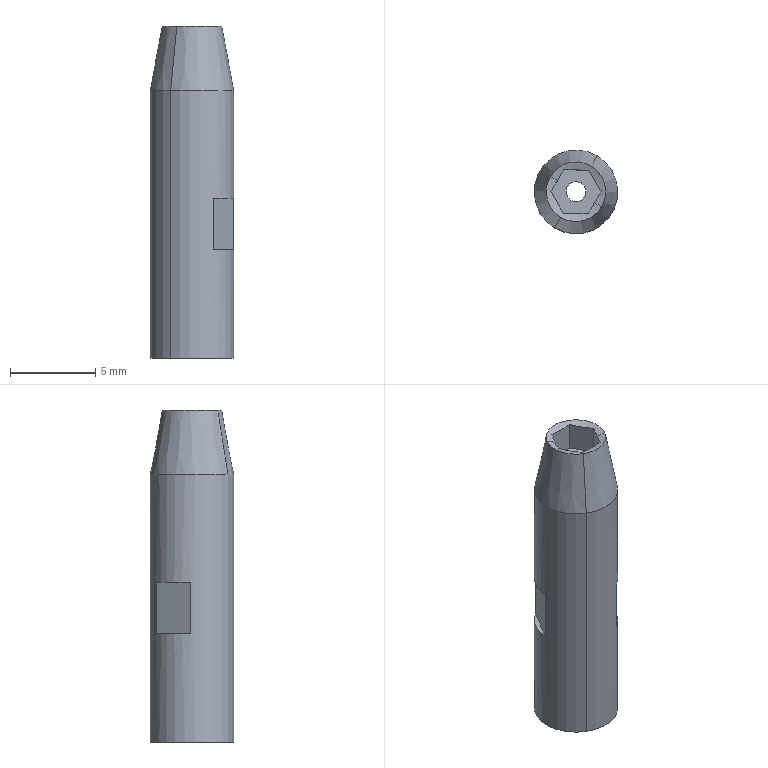Component | SolidWorks | PointedHead-2 | 1 solid | 24 faces | box 4.9 x 4.9 x 19.5 mm | volume 169 mm3 | plane 14 | cone 4 | cylinder 4 | sphere 2 | commonest cylinder face diameters 3.5 x2 4.9 x2
build123d program:
from build123d import *

# Parameters (mm, degrees)
SKETCH1_R                      = 2.45
EXTRUDE1_DEPTH                 = 19.5
CHAMFER1_SIZE                  = 0.7
CHAMFER1_SIZE2                 = 3.8
F_3_5_3_5_DIAMETER_HOLE1_D     = 3.5
F_3_5_3_5_DIAMETER_HOLE1_DEPTH = 17
F_3_5_3_5_DIAMETER_HOLE1_TIP   = 1.052
CUT_EXTRUDE1_DEPTH             = 1.8
CUT_EXTRUDE2_DEPTH             = 20.805
CUT_EXTRUDE2_DEPTH_BACK        = 20.805
SKETCH6_W                      = 3
SKETCH6_H                      = 0.3


with BuildPart() as part:
    # Sketch1 → Extrude1 (new body)
    with BuildSketch(Plane(origin=(0, 0, 0), x_dir=(0, 0, -1), z_dir=(1, 0, 0))):
        Circle(SKETCH1_R)
    extrude(amount=EXTRUDE1_DEPTH)

    # Chamfer1
    chamfer1_edges = [part.edges().sort_by_distance(p)[0] for p in [
        (0, 0, 2.45),
    ]]
    chamfer1_side = [part.faces().sort_by_distance(p)[0] for p in [
        (0, 0, 0),
    ]]
    chamfer(chamfer1_edges, length=CHAMFER1_SIZE, length2=CHAMFER1_SIZE2, reference=chamfer1_side[0])

    # 3.5 _3.5_ Diameter Hole1
    with Locations(Plane(origin=(19.5, 0, 0), x_dir=(0, 0, -1), z_dir=(1, 0, 0))):
        with Locations((0, 0)):
            Hole(F_3_5_3_5_DIAMETER_HOLE1_D / 2, depth=F_3_5_3_5_DIAMETER_HOLE1_DEPTH)
            with Locations((0, 0, -(F_3_5_3_5_DIAMETER_HOLE1_DEPTH + F_3_5_3_5_DIAMETER_HOLE1_TIP / 2))):  # 118° drill point
                Cone(0, F_3_5_3_5_DIAMETER_HOLE1_D / 2, F_3_5_3_5_DIAMETER_HOLE1_TIP, mode=Mode.SUBTRACT)

    # Sketch4 → Cut-Extrude1 (cut)
    with BuildSketch(Plane.ZY):
        Polygon((1.472, 0), (0.7361, 1.275), (-0.7361, 1.275), (-1.472, 0), (-0.7361, -1.275), (0.7361, -1.275), align=None)
    extrude(amount=-CUT_EXTRUDE1_DEPTH, mode=Mode.SUBTRACT)

    # Sketch5 → Cut-Revolve2 (revolve, cut)
    with BuildSketch(Plane.XY, mode=Mode.PRIVATE) as cut_revolve2_sk:
        with BuildLine():
            Line((0, 1.75), (0, 0))
            Line((0, 0), (0.3163, 0))
            ThreePointArc((0.3163, 0), (0.2366, 0.8892), (0, 1.75))
        make_face()
    revolve(cut_revolve2_sk.sketch.rotate(Axis((0, 0, 0), (-1, 0, 0)), 90), axis=Axis((0, 0, 0), (-1, 0, 0)), mode=Mode.SUBTRACT)

    # Sketch6 → Cut-Extrude2 (cut, two sides: drawn at the far end of the back side and taken through both)
    with BuildSketch(Plane.XY.offset(-CUT_EXTRUDE2_DEPTH_BACK)):
        with Locations((11.65, 2.3)):
            Rectangle(SKETCH6_W, SKETCH6_H)
        with Locations((11.65, -2.3)):
            Rectangle(SKETCH6_W, SKETCH6_H)
    extrude(amount=CUT_EXTRUDE2_DEPTH + CUT_EXTRUDE2_DEPTH_BACK, mode=Mode.SUBTRACT)


solid = part.part

# Placed as in the assembly
solid = solid.moved(Location((22.667, 79.622, -18.387), (90, -30.736, -90)))
STEP:
#1=CARTESIAN_POINT('',(0.8332,3.17,-0.7239));
#2=VERTEX_POINT('',#1);
#3=CARTESIAN_POINT('',(0.9276,3.194,-0.7239));
#4=VERTEX_POINT('',#3);
#5=CARTESIAN_POINT('',(0.8924,3.135,-0.7239));
#6=DIRECTION('',(-0.,0.,-1.));
#7=DIRECTION('',(-0.8595,0.5111,0.));
#8=AXIS2_PLACEMENT_3D('',#5,#6,#7);
#9=CIRCLE('',#8,0.0689);
#10=EDGE_CURVE('',#2,#4,#9,.T.);
#11=ORIENTED_EDGE('',*,*,#10,.F.);
#12=CARTESIAN_POINT('',(0.8493,3.16,-0.7298));
#13=VERTEX_POINT('',#12);
#14=CARTESIAN_POINT('',(0.8924,3.135,-0.5395));
#15=DIRECTION('',(-0.5111,-0.8595,0.));
#16=DIRECTION('',(0.8595,-0.5111,0.));
#17=AXIS2_PLACEMENT_3D('',#14,#15,#16);
#18=CIRCLE('',#17,0.1969);
#19=EDGE_CURVE('',#2,#13,#18,.T.);
#20=ORIENTED_EDGE('',*,*,#19,.T.);
#21=CARTESIAN_POINT('',(0.8641,3.185,-0.7276));
#22=VERTEX_POINT('',#21);
#23=CARTESIAN_POINT('',(0.8493,3.16,-0.5395));
#24=DIRECTION('',(-0.8595,0.5111,0.));
#25=DIRECTION('',(0.5111,0.8595,0.));
#26=AXIS2_PLACEMENT_3D('',#23,#24,#25);
#27=CIRCLE('',#26,0.1903);
#28=EDGE_CURVE('',#22,#13,#27,.T.);
#29=ORIENTED_EDGE('',*,*,#28,.F.);
#30=CARTESIAN_POINT('',(0.922,3.185,-0.7276));
#31=VERTEX_POINT('',#30);
#32=CARTESIAN_POINT('',(0.893,3.185,-0.5395));
#33=DIRECTION('',(0.01285,0.9999,-0.));
#34=DIRECTION('',(0.9999,-0.01285,-0.));
#35=AXIS2_PLACEMENT_3D('',#32,#33,#34);
#36=CIRCLE('',#35,0.1903);
#37=EDGE_CURVE('',#31,#22,#36,.T.);
#38=ORIENTED_EDGE('',*,*,#37,.F.);
#39=CARTESIAN_POINT('',(0.9504,3.134,-0.7276));
#40=VERTEX_POINT('',#39);
#41=CARTESIAN_POINT('',(0.9362,3.159,-0.5395));
#42=DIRECTION('',(0.8724,0.4888,-0.));
#43=DIRECTION('',(0.4888,-0.8724,0.));
#44=AXIS2_PLACEMENT_3D('',#41,#42,#43);
#45=CIRCLE('',#44,0.1903);
#46=EDGE_CURVE('',#40,#31,#45,.T.);
#47=ORIENTED_EDGE('',*,*,#46,.F.);
#48=CARTESIAN_POINT('',(0.9355,3.109,-0.7298));
#49=VERTEX_POINT('',#48);
#50=CARTESIAN_POINT('',(0.9355,3.109,-0.5395));
#51=DIRECTION('',(0.8595,-0.5111,-0.));
#52=DIRECTION('',(-0.5111,-0.8595,0.));
#53=AXIS2_PLACEMENT_3D('',#50,#51,#52);
#54=CIRCLE('',#53,0.1903);
#55=EDGE_CURVE('',#49,#40,#54,.T.);
#56=ORIENTED_EDGE('',*,*,#55,.F.);
#57=CARTESIAN_POINT('',(0.9516,3.1,-0.7239));
#58=VERTEX_POINT('',#57);
#59=CARTESIAN_POINT('',(0.8924,3.135,-0.5395));
#60=DIRECTION('',(0.5111,0.8595,-0.));
#61=DIRECTION('',(-0.8595,0.5111,0.));
#62=AXIS2_PLACEMENT_3D('',#59,#60,#61);
#63=CIRCLE('',#62,0.1969);
#64=EDGE_CURVE('',#58,#49,#63,.T.);
#65=ORIENTED_EDGE('',*,*,#64,.F.);
#66=CARTESIAN_POINT('',(0.8924,3.135,-0.7239));
#67=DIRECTION('',(-0.,0.,-1.));
#68=DIRECTION('',(-0.8595,0.5111,0.));
#69=AXIS2_PLACEMENT_3D('',#66,#67,#68);
#70=CIRCLE('',#69,0.0689);
#71=EDGE_CURVE('',#4,#58,#70,.T.);
#72=ORIENTED_EDGE('',*,*,#71,.F.);
#73=EDGE_LOOP('',(#11,#20,#29,#38,#47,#56,#65,#72));
#74=FACE_OUTER_BOUND('',#73,.T.);
#75=CARTESIAN_POINT('',(0.8924,3.135,-0.5395));
#76=DIRECTION('',(-0.5111,-0.8595,0.));
#77=DIRECTION('',(0.8595,-0.5111,-0.));
#78=AXIS2_PLACEMENT_3D('',#75,#76,#77);
#79=SPHERICAL_SURFACE('',#78,0.1969);
#80=ADVANCED_FACE('',(#74),#79,.F.);
#81=CARTESIAN_POINT('',(0.8806,3.115,-0.7948));
#82=VERTEX_POINT('',#81);
#83=CARTESIAN_POINT('',(0.9042,3.155,-0.7948));
#84=VERTEX_POINT('',#83);
#85=CARTESIAN_POINT('',(0.8924,3.135,-0.7948));
#86=DIRECTION('',(0.,-0.,1.));
#87=DIRECTION('',(-0.5111,-0.8595,0.));
#88=AXIS2_PLACEMENT_3D('',#85,#86,#87);
#89=CIRCLE('',#88,0.02303);
#90=EDGE_CURVE('',#82,#84,#89,.T.);
#91=ORIENTED_EDGE('',*,*,#90,.T.);
#92=CARTESIAN_POINT('',(0.9276,3.194,-0.8223));
#93=VERTEX_POINT('',#92);
#94=CARTESIAN_POINT('',(0.9276,3.194,-0.8223));
#95=DIRECTION('',(0.4381,0.7368,-0.515));
#96=VECTOR('',#95,39.37);
#97=LINE('',#94,#96);
#98=EDGE_CURVE('',#84,#93,#97,.T.);
#99=ORIENTED_EDGE('',*,*,#98,.T.);
#100=CARTESIAN_POINT('',(0.8572,3.076,-0.8223));
#101=VERTEX_POINT('',#100);
#102=CARTESIAN_POINT('',(0.8924,3.135,-0.8223));
#103=DIRECTION('',(-0.,0.,-1.));
#104=DIRECTION('',(-0.5111,-0.8595,0.));
#105=AXIS2_PLACEMENT_3D('',#102,#103,#104);
#106=CIRCLE('',#105,0.0689);
#107=EDGE_CURVE('',#93,#101,#106,.T.);
#108=ORIENTED_EDGE('',*,*,#107,.T.);
#109=CARTESIAN_POINT('',(0.8572,3.076,-0.8223));
#110=DIRECTION('',(-0.4381,-0.7368,-0.515));
#111=VECTOR('',#110,39.37);
#112=LINE('',#109,#111);
#113=EDGE_CURVE('',#82,#101,#112,.T.);
#114=ORIENTED_EDGE('',*,*,#113,.F.);
#115=EDGE_LOOP('',(#91,#99,#108,#114));
#116=FACE_OUTER_BOUND('',#115,.T.);
#117=CARTESIAN_POINT('',(0.8924,3.135,-0.8223));
#118=DIRECTION('',(-0.,0.,-1.));
#119=DIRECTION('',(-0.5111,-0.8595,0.));
#120=AXIS2_PLACEMENT_3D('',#117,#118,#119);
#121=CONICAL_SURFACE('',#120,0.0689,1.03);
#122=ADVANCED_FACE('',(#116),#121,.F.);
#123=ORIENTED_EDGE('',*,*,#107,.F.);
#124=CARTESIAN_POINT('',(0.9276,3.194,-1.492));
#125=VERTEX_POINT('',#124);
#126=CARTESIAN_POINT('',(0.9276,3.194,-1.492));
#127=DIRECTION('',(-0.,0.,-1.));
#128=VECTOR('',#127,39.37);
#129=LINE('',#126,#128);
#130=EDGE_CURVE('',#93,#125,#129,.T.);
#131=ORIENTED_EDGE('',*,*,#130,.T.);
#132=CARTESIAN_POINT('',(0.8572,3.076,-1.492));
#133=VERTEX_POINT('',#132);
#134=CARTESIAN_POINT('',(0.8924,3.135,-1.492));
#135=DIRECTION('',(-0.,0.,-1.));
#136=DIRECTION('',(-0.5111,-0.8595,0.));
#137=AXIS2_PLACEMENT_3D('',#134,#135,#136);
#138=CIRCLE('',#137,0.0689);
#139=EDGE_CURVE('',#125,#133,#138,.T.);
#140=ORIENTED_EDGE('',*,*,#139,.T.);
#141=CARTESIAN_POINT('',(0.8572,3.076,-1.492));
#142=DIRECTION('',(-0.,0.,-1.));
#143=VECTOR('',#142,39.37);
#144=LINE('',#141,#143);
#145=EDGE_CURVE('',#101,#133,#144,.T.);
#146=ORIENTED_EDGE('',*,*,#145,.F.);
#147=EDGE_LOOP('',(#123,#131,#140,#146));
#148=FACE_OUTER_BOUND('',#147,.T.);
#149=CARTESIAN_POINT('',(0.8924,3.135,-1.492));
#150=DIRECTION('',(-0.,0.,-1.));
#151=DIRECTION('',(-0.5111,-0.8595,0.));
#152=AXIS2_PLACEMENT_3D('',#149,#150,#151);
#153=CYLINDRICAL_SURFACE('',#152,0.0689);
#154=ADVANCED_FACE('',(#148),#153,.F.);
#155=CARTESIAN_POINT('',(0.8572,3.076,-0.7239));
#156=VERTEX_POINT('',#155);
#157=CARTESIAN_POINT('',(0.8924,3.135,-0.7239));
#158=DIRECTION('',(-0.,0.,-1.));
#159=DIRECTION('',(-0.8595,0.5111,0.));
#160=AXIS2_PLACEMENT_3D('',#157,#158,#159);
#161=CIRCLE('',#160,0.0689);
#162=EDGE_CURVE('',#156,#2,#161,.T.);
#163=ORIENTED_EDGE('',*,*,#162,.T.);
#164=ORIENTED_EDGE('',*,*,#10,.T.);
#165=CARTESIAN_POINT('',(0.9417,3.218,-0.8735));
#166=VERTEX_POINT('',#165);
#167=CARTESIAN_POINT('',(0.9417,3.218,-0.8735));
#168=DIRECTION('',(0.09259,0.1557,-0.9835));
#169=VECTOR('',#168,39.37);
#170=LINE('',#167,#169);
#171=EDGE_CURVE('',#4,#166,#170,.T.);
#172=ORIENTED_EDGE('',*,*,#171,.T.);
#173=CARTESIAN_POINT('',(0.8431,3.052,-0.8735));
#174=VERTEX_POINT('',#173);
#175=CARTESIAN_POINT('',(0.8924,3.135,-0.8735));
#176=DIRECTION('',(-0.,0.,-1.));
#177=DIRECTION('',(-0.5111,-0.8595,0.));
#178=AXIS2_PLACEMENT_3D('',#175,#176,#177);
#179=CIRCLE('',#178,0.09646);
#180=EDGE_CURVE('',#174,#166,#179,.T.);
#181=ORIENTED_EDGE('',*,*,#180,.F.);
#182=CARTESIAN_POINT('',(0.8431,3.052,-0.8735));
#183=DIRECTION('',(-0.09259,-0.1557,-0.9835));
#184=VECTOR('',#183,39.37);
#185=LINE('',#182,#184);
#186=EDGE_CURVE('',#156,#174,#185,.T.);
#187=ORIENTED_EDGE('',*,*,#186,.F.);
#188=EDGE_LOOP('',(#163,#164,#172,#181,#187));
#189=FACE_OUTER_BOUND('',#188,.T.);
#190=CARTESIAN_POINT('',(0.8924,3.135,-0.8735));
#191=DIRECTION('',(-0.,0.,-1.));
#192=DIRECTION('',(-0.5111,-0.8595,0.));
#193=AXIS2_PLACEMENT_3D('',#190,#191,#192);
#194=CONICAL_SURFACE('',#193,0.09646,0.1822);
#195=ADVANCED_FACE('',(#189),#194,.T.);
#196=CARTESIAN_POINT('',(0.796,3.138,-1.242));
#197=VERTEX_POINT('',#196);
#198=CARTESIAN_POINT('',(0.8433,3.218,-1.242));
#199=VERTEX_POINT('',#198);
#200=CARTESIAN_POINT('',(0.8924,3.135,-1.242));
#201=DIRECTION('',(-0.,0.,-1.));
#202=DIRECTION('',(-0.5111,-0.8595,0.));
#203=AXIS2_PLACEMENT_3D('',#200,#201,#202);
#204=CIRCLE('',#203,0.09646);
#205=EDGE_CURVE('',#197,#199,#204,.T.);
#206=ORIENTED_EDGE('',*,*,#205,.T.);
#207=CARTESIAN_POINT('',(0.8433,3.218,-1.123));
#208=VERTEX_POINT('',#207);
#209=CARTESIAN_POINT('',(0.8433,3.218,-1.492));
#210=DIRECTION('',(0.,-0.,1.));
#211=VECTOR('',#210,39.37);
#212=LINE('',#209,#211);
#213=EDGE_CURVE('',#199,#208,#212,.T.);
#214=ORIENTED_EDGE('',*,*,#213,.T.);
#215=CARTESIAN_POINT('',(0.796,3.138,-1.123));
#216=VERTEX_POINT('',#215);
#217=CARTESIAN_POINT('',(0.8924,3.135,-1.123));
#218=DIRECTION('',(0.,-0.,1.));
#219=DIRECTION('',(0.5111,0.8595,0.));
#220=AXIS2_PLACEMENT_3D('',#217,#218,#219);
#221=CIRCLE('',#220,0.09646);
#222=EDGE_CURVE('',#208,#216,#221,.T.);
#223=ORIENTED_EDGE('',*,*,#222,.T.);
#224=CARTESIAN_POINT('',(0.796,3.138,-1.492));
#225=DIRECTION('',(-0.,0.,-1.));
#226=VECTOR('',#225,39.37);
#227=LINE('',#224,#226);
#228=EDGE_CURVE('',#216,#197,#227,.T.);
#229=ORIENTED_EDGE('',*,*,#228,.T.);
#230=EDGE_LOOP('',(#206,#214,#223,#229));
#231=FACE_BOUND('',#230,.T.);
#232=CARTESIAN_POINT('',(0.8431,3.052,-1.492));
#233=VERTEX_POINT('',#232);
#234=CARTESIAN_POINT('',(0.9417,3.218,-1.492));
#235=VERTEX_POINT('',#234);
#236=CARTESIAN_POINT('',(0.8924,3.135,-1.492));
#237=DIRECTION('',(-0.,0.,-1.));
#238=DIRECTION('',(-0.5111,-0.8595,0.));
#239=AXIS2_PLACEMENT_3D('',#236,#237,#238);
#240=CIRCLE('',#239,0.09646);
#241=EDGE_CURVE('',#233,#235,#240,.T.);
#242=ORIENTED_EDGE('',*,*,#241,.F.);
#243=CARTESIAN_POINT('',(0.8431,3.052,-1.492));
#244=DIRECTION('',(0.,-0.,1.));
#245=VECTOR('',#244,39.37);
#246=LINE('',#243,#245);
#247=EDGE_CURVE('',#233,#174,#246,.T.);
#248=ORIENTED_EDGE('',*,*,#247,.T.);
#249=ORIENTED_EDGE('',*,*,#180,.T.);
#250=CARTESIAN_POINT('',(0.9417,3.218,-1.492));
#251=DIRECTION('',(0.,-0.,1.));
#252=VECTOR('',#251,39.37);
#253=LINE('',#250,#252);
#254=EDGE_CURVE('',#235,#166,#253,.T.);
#255=ORIENTED_EDGE('',*,*,#254,.F.);
#256=EDGE_LOOP('',(#242,#248,#249,#255));
#257=FACE_OUTER_BOUND('',#256,.T.);
#258=CARTESIAN_POINT('',(0.8924,3.135,-1.492));
#259=DIRECTION('',(0.,-0.,1.));
#260=DIRECTION('',(0.5111,0.8595,0.));
#261=AXIS2_PLACEMENT_3D('',#258,#259,#260);
#262=CYLINDRICAL_SURFACE('',#261,0.09646);
#263=ADVANCED_FACE('',(#231,#257),#262,.T.);
#264=ORIENTED_EDGE('',*,*,#247,.F.);
#265=CARTESIAN_POINT('',(0.8924,3.135,-1.492));
#266=DIRECTION('',(-0.,0.,-1.));
#267=DIRECTION('',(-0.5111,-0.8595,0.));
#268=AXIS2_PLACEMENT_3D('',#265,#266,#267);
#269=CIRCLE('',#268,0.09646);
#270=EDGE_CURVE('',#235,#233,#269,.T.);
#271=ORIENTED_EDGE('',*,*,#270,.F.);
#272=ORIENTED_EDGE('',*,*,#254,.T.);
#273=CARTESIAN_POINT('',(0.8924,3.135,-0.8735));
#274=DIRECTION('',(-0.,0.,-1.));
#275=DIRECTION('',(-0.5111,-0.8595,0.));
#276=AXIS2_PLACEMENT_3D('',#273,#274,#275);
#277=CIRCLE('',#276,0.09646);
#278=EDGE_CURVE('',#166,#174,#277,.T.);
#279=ORIENTED_EDGE('',*,*,#278,.T.);
#280=EDGE_LOOP('',(#264,#271,#272,#279));
#281=FACE_OUTER_BOUND('',#280,.T.);
#282=CARTESIAN_POINT('',(0.9888,3.131,-1.123));
#283=VERTEX_POINT('',#282);
#284=CARTESIAN_POINT('',(0.9888,3.131,-1.242));
#285=VERTEX_POINT('',#284);
#286=CARTESIAN_POINT('',(0.9888,3.131,-1.492));
#287=DIRECTION('',(-0.,0.,-1.));
#288=VECTOR('',#287,39.37);
#289=LINE('',#286,#288);
#290=EDGE_CURVE('',#283,#285,#289,.T.);
#291=ORIENTED_EDGE('',*,*,#290,.T.);
#292=CARTESIAN_POINT('',(0.9415,3.052,-1.242));
#293=VERTEX_POINT('',#292);
#294=CARTESIAN_POINT('',(0.8924,3.135,-1.242));
#295=DIRECTION('',(-0.,0.,-1.));
#296=DIRECTION('',(-0.8595,0.5111,0.));
#297=AXIS2_PLACEMENT_3D('',#294,#295,#296);
#298=CIRCLE('',#297,0.09646);
#299=EDGE_CURVE('',#285,#293,#298,.T.);
#300=ORIENTED_EDGE('',*,*,#299,.T.);
#301=CARTESIAN_POINT('',(0.9415,3.052,-1.123));
#302=VERTEX_POINT('',#301);
#303=CARTESIAN_POINT('',(0.9415,3.052,-1.492));
#304=DIRECTION('',(0.,-0.,1.));
#305=VECTOR('',#304,39.37);
#306=LINE('',#303,#305);
#307=EDGE_CURVE('',#293,#302,#306,.T.);
#308=ORIENTED_EDGE('',*,*,#307,.T.);
#309=CARTESIAN_POINT('',(0.8924,3.135,-1.123));
#310=DIRECTION('',(-0.,0.,1.));
#311=DIRECTION('',(0.8595,-0.5111,0.));
#312=AXIS2_PLACEMENT_3D('',#309,#310,#311);
#313=CIRCLE('',#312,0.09646);
#314=EDGE_CURVE('',#302,#283,#313,.T.);
#315=ORIENTED_EDGE('',*,*,#314,.T.);
#316=EDGE_LOOP('',(#291,#300,#308,#315));
#317=FACE_BOUND('',#316,.T.);
#318=CARTESIAN_POINT('',(0.8924,3.135,-1.492));
#319=DIRECTION('',(0.,-0.,1.));
#320=DIRECTION('',(0.5111,0.8595,0.));
#321=AXIS2_PLACEMENT_3D('',#318,#319,#320);
#322=CYLINDRICAL_SURFACE('',#321,0.09646);
#323=ADVANCED_FACE('',(#281,#317),#322,.T.);
#324=CARTESIAN_POINT('',(0.8924,3.135,-1.492));
#325=DIRECTION('',(-0.,0.,-1.));
#326=DIRECTION('',(-0.5111,-0.8595,0.));
#327=AXIS2_PLACEMENT_3D('',#324,#325,#326);
#328=CIRCLE('',#327,0.0689);
#329=EDGE_CURVE('',#133,#125,#328,.T.);
#330=ORIENTED_EDGE('',*,*,#329,.F.);
#331=ORIENTED_EDGE('',*,*,#139,.F.);
#332=EDGE_LOOP('',(#330,#331));
#333=FACE_BOUND('',#332,.T.);
#334=ORIENTED_EDGE('',*,*,#270,.T.);
#335=ORIENTED_EDGE('',*,*,#241,.T.);
#336=EDGE_LOOP('',(#334,#335));
#337=FACE_OUTER_BOUND('',#336,.T.);
#338=CARTESIAN_POINT('',(0.8924,3.135,-1.492));
#339=DIRECTION('',(-0.,0.,-1.));
#340=DIRECTION('',(-0.5111,-0.8595,0.));
#341=AXIS2_PLACEMENT_3D('',#338,#339,#340);
#342=PLANE('',#341);
#343=ADVANCED_FACE('',(#333,#337),#342,.T.);
#344=ORIENTED_EDGE('',*,*,#171,.F.);
#345=ORIENTED_EDGE('',*,*,#71,.T.);
#346=CARTESIAN_POINT('',(0.8924,3.135,-0.7239));
#347=DIRECTION('',(-0.,0.,-1.));
#348=DIRECTION('',(-0.8595,0.5111,0.));
#349=AXIS2_PLACEMENT_3D('',#346,#347,#348);
#350=CIRCLE('',#349,0.0689);
#351=EDGE_CURVE('',#58,#156,#350,.T.);
#352=ORIENTED_EDGE('',*,*,#351,.T.);
#353=ORIENTED_EDGE('',*,*,#186,.T.);
#354=ORIENTED_EDGE('',*,*,#278,.F.);
#355=EDGE_LOOP('',(#344,#345,#352,#353,#354));
#356=FACE_OUTER_BOUND('',#355,.T.);
#357=CARTESIAN_POINT('',(0.8924,3.135,-0.8735));
#358=DIRECTION('',(-0.,0.,-1.));
#359=DIRECTION('',(-0.5111,-0.8595,0.));
#360=AXIS2_PLACEMENT_3D('',#357,#358,#359);
#361=CONICAL_SURFACE('',#360,0.09646,0.1822);
#362=ADVANCED_FACE('',(#356),#361,.T.);
#363=ORIENTED_EDGE('',*,*,#130,.F.);
#364=CARTESIAN_POINT('',(0.8924,3.135,-0.8223));
#365=DIRECTION('',(-0.,0.,-1.));
#366=DIRECTION('',(-0.5111,-0.8595,0.));
#367=AXIS2_PLACEMENT_3D('',#364,#365,#366);
#368=CIRCLE('',#367,0.0689);
#369=EDGE_CURVE('',#101,#93,#368,.T.);
#370=ORIENTED_EDGE('',*,*,#369,.F.);
#371=ORIENTED_EDGE('',*,*,#145,.T.);
#372=ORIENTED_EDGE('',*,*,#329,.T.);
#373=EDGE_LOOP('',(#363,#370,#371,#372));
#374=FACE_OUTER_BOUND('',#373,.T.);
#375=CARTESIAN_POINT('',(0.8924,3.135,-1.492));
#376=DIRECTION('',(-0.,0.,-1.));
#377=DIRECTION('',(-0.5111,-0.8595,0.));
#378=AXIS2_PLACEMENT_3D('',#375,#376,#377);
#379=CYLINDRICAL_SURFACE('',#378,0.0689);
#380=ADVANCED_FACE('',(#374),#379,.F.);
#381=ORIENTED_EDGE('',*,*,#98,.F.);
#382=CARTESIAN_POINT('',(0.8924,3.135,-0.7948));
#383=DIRECTION('',(0.,-0.,1.));
#384=DIRECTION('',(-0.5111,-0.8595,0.));
#385=AXIS2_PLACEMENT_3D('',#382,#383,#384);
#386=CIRCLE('',#385,0.02303);
#387=EDGE_CURVE('',#84,#82,#386,.T.);
#388=ORIENTED_EDGE('',*,*,#387,.T.);
#389=ORIENTED_EDGE('',*,*,#113,.T.);
#390=ORIENTED_EDGE('',*,*,#369,.T.);
#391=EDGE_LOOP('',(#381,#388,#389,#390));
#392=FACE_OUTER_BOUND('',#391,.T.);
#393=CARTESIAN_POINT('',(0.8924,3.135,-0.8223));
#394=DIRECTION('',(-0.,0.,-1.));
#395=DIRECTION('',(-0.5111,-0.8595,0.));
#396=AXIS2_PLACEMENT_3D('',#393,#394,#395);
#397=CONICAL_SURFACE('',#396,0.0689,1.03);
#398=ADVANCED_FACE('',(#392),#397,.F.);
#399=CARTESIAN_POINT('',(0.9504,3.134,-0.7948));
#400=VERTEX_POINT('',#399);
#401=CARTESIAN_POINT('',(0.922,3.185,-0.7948));
#402=VERTEX_POINT('',#401);
#403=CARTESIAN_POINT('',(0.9504,3.134,-0.7948));
#404=DIRECTION('',(-0.4888,0.8724,0.));
#405=VECTOR('',#404,39.37);
#406=LINE('',#403,#405);
#407=EDGE_CURVE('',#400,#402,#406,.T.);
#408=ORIENTED_EDGE('',*,*,#407,.T.);
#409=CARTESIAN_POINT('',(0.8641,3.185,-0.7948));
#410=VERTEX_POINT('',#409);
#411=CARTESIAN_POINT('',(0.922,3.185,-0.7948));
#412=DIRECTION('',(-0.9999,0.01285,0.));
#413=VECTOR('',#412,39.37);
#414=LINE('',#411,#413);
#415=EDGE_CURVE('',#402,#410,#414,.T.);
#416=ORIENTED_EDGE('',*,*,#415,.T.);
#417=CARTESIAN_POINT('',(0.8344,3.135,-0.7948));
#418=VERTEX_POINT('',#417);
#419=CARTESIAN_POINT('',(0.8641,3.185,-0.7948));
#420=DIRECTION('',(-0.5111,-0.8595,0.));
#421=VECTOR('',#420,39.37);
#422=LINE('',#419,#421);
#423=EDGE_CURVE('',#410,#418,#422,.T.);
#424=ORIENTED_EDGE('',*,*,#423,.T.);
#425=CARTESIAN_POINT('',(0.8628,3.085,-0.7948));
#426=VERTEX_POINT('',#425);
#427=CARTESIAN_POINT('',(0.8344,3.135,-0.7948));
#428=DIRECTION('',(0.4888,-0.8724,-0.));
#429=VECTOR('',#428,39.37);
#430=LINE('',#427,#429);
#431=EDGE_CURVE('',#418,#426,#430,.T.);
#432=ORIENTED_EDGE('',*,*,#431,.T.);
#433=CARTESIAN_POINT('',(0.9207,3.084,-0.7948));
#434=VERTEX_POINT('',#433);
#435=CARTESIAN_POINT('',(0.8628,3.085,-0.7948));
#436=DIRECTION('',(0.9999,-0.01285,-0.));
#437=VECTOR('',#436,39.37);
#438=LINE('',#435,#437);
#439=EDGE_CURVE('',#426,#434,#438,.T.);
#440=ORIENTED_EDGE('',*,*,#439,.T.);
#441=CARTESIAN_POINT('',(0.9207,3.084,-0.7948));
#442=DIRECTION('',(0.5111,0.8595,-0.));
#443=VECTOR('',#442,39.37);
#444=LINE('',#441,#443);
#445=EDGE_CURVE('',#434,#400,#444,.T.);
#446=ORIENTED_EDGE('',*,*,#445,.T.);
#447=EDGE_LOOP('',(#408,#416,#424,#432,#440,#446));
#448=FACE_OUTER_BOUND('',#447,.T.);
#449=ORIENTED_EDGE('',*,*,#90,.F.);
#450=ORIENTED_EDGE('',*,*,#387,.F.);
#451=EDGE_LOOP('',(#449,#450));
#452=FACE_BOUND('',#451,.T.);
#453=CARTESIAN_POINT('',(0.9504,3.134,-0.7948));
#454=DIRECTION('',(-0.,0.,-1.));
#455=DIRECTION('',(-0.5111,-0.8595,0.));
#456=AXIS2_PLACEMENT_3D('',#453,#454,#455);
#457=PLANE('',#456);
#458=ADVANCED_FACE('',(#448,#452),#457,.F.);
#459=CARTESIAN_POINT('',(0.9504,3.134,-0.7948));
#460=DIRECTION('',(0.,-0.,1.));
#461=VECTOR('',#460,39.37);
#462=LINE('',#459,#461);
#463=EDGE_CURVE('',#400,#40,#462,.T.);
#464=ORIENTED_EDGE('',*,*,#463,.T.);
#465=ORIENTED_EDGE('',*,*,#46,.T.);
#466=CARTESIAN_POINT('',(0.922,3.185,-0.7948));
#467=DIRECTION('',(0.,-0.,1.));
#468=VECTOR('',#467,39.37);
#469=LINE('',#466,#468);
#470=EDGE_CURVE('',#402,#31,#469,.T.);
#471=ORIENTED_EDGE('',*,*,#470,.F.);
#472=ORIENTED_EDGE('',*,*,#407,.F.);
#473=EDGE_LOOP('',(#464,#465,#471,#472));
#474=FACE_OUTER_BOUND('',#473,.T.);
#475=CARTESIAN_POINT('',(0.9504,3.134,-0.7948));
#476=DIRECTION('',(0.8724,0.4888,-0.));
#477=DIRECTION('',(0.4888,-0.8724,-0.));
#478=AXIS2_PLACEMENT_3D('',#475,#476,#477);
#479=PLANE('',#478);
#480=ADVANCED_FACE('',(#474),#479,.F.);
#481=CARTESIAN_POINT('',(0.9207,3.084,-0.7276));
#482=VERTEX_POINT('',#481);
#483=CARTESIAN_POINT('',(0.9207,3.084,-0.7948));
#484=DIRECTION('',(0.,-0.,1.));
#485=VECTOR('',#484,39.37);
#486=LINE('',#483,#485);
#487=EDGE_CURVE('',#434,#482,#486,.T.);
#488=ORIENTED_EDGE('',*,*,#487,.T.);
#489=CARTESIAN_POINT('',(0.9355,3.109,-0.5395));
#490=DIRECTION('',(0.8595,-0.5111,-0.));
#491=DIRECTION('',(-0.5111,-0.8595,0.));
#492=AXIS2_PLACEMENT_3D('',#489,#490,#491);
#493=CIRCLE('',#492,0.1903);
#494=EDGE_CURVE('',#482,#49,#493,.T.);
#495=ORIENTED_EDGE('',*,*,#494,.T.);
#496=ORIENTED_EDGE('',*,*,#55,.T.);
#497=ORIENTED_EDGE('',*,*,#463,.F.);
#498=ORIENTED_EDGE('',*,*,#445,.F.);
#499=EDGE_LOOP('',(#488,#495,#496,#497,#498));
#500=FACE_OUTER_BOUND('',#499,.T.);
#501=CARTESIAN_POINT('',(0.9207,3.084,-0.7948));
#502=DIRECTION('',(0.8595,-0.5111,-0.));
#503=DIRECTION('',(-0.5111,-0.8595,0.));
#504=AXIS2_PLACEMENT_3D('',#501,#502,#503);
#505=PLANE('',#504);
#506=ADVANCED_FACE('',(#500),#505,.F.);
#507=CARTESIAN_POINT('',(0.8628,3.085,-0.7276));
#508=VERTEX_POINT('',#507);
#509=CARTESIAN_POINT('',(0.8628,3.085,-0.7948));
#510=DIRECTION('',(0.,-0.,1.));
#511=VECTOR('',#510,39.37);
#512=LINE('',#509,#511);
#513=EDGE_CURVE('',#426,#508,#512,.T.);
#514=ORIENTED_EDGE('',*,*,#513,.T.);
#515=CARTESIAN_POINT('',(0.8918,3.085,-0.5395));
#516=DIRECTION('',(-0.01285,-0.9999,0.));
#517=DIRECTION('',(-0.9999,0.01285,0.));
#518=AXIS2_PLACEMENT_3D('',#515,#516,#517);
#519=CIRCLE('',#518,0.1903);
#520=EDGE_CURVE('',#508,#482,#519,.T.);
#521=ORIENTED_EDGE('',*,*,#520,.T.);
#522=ORIENTED_EDGE('',*,*,#487,.F.);
#523=ORIENTED_EDGE('',*,*,#439,.F.);
#524=EDGE_LOOP('',(#514,#521,#522,#523));
#525=FACE_OUTER_BOUND('',#524,.T.);
#526=CARTESIAN_POINT('',(0.8628,3.085,-0.7948));
#527=DIRECTION('',(-0.01285,-0.9999,0.));
#528=DIRECTION('',(-0.9999,0.01285,0.));
#529=AXIS2_PLACEMENT_3D('',#526,#527,#528);
#530=PLANE('',#529);
#531=ADVANCED_FACE('',(#525),#530,.F.);
#532=CARTESIAN_POINT('',(0.8344,3.135,-0.7276));
#533=VERTEX_POINT('',#532);
#534=CARTESIAN_POINT('',(0.8344,3.135,-0.7948));
#535=DIRECTION('',(0.,-0.,1.));
#536=VECTOR('',#535,39.37);
#537=LINE('',#534,#536);
#538=EDGE_CURVE('',#418,#533,#537,.T.);
#539=ORIENTED_EDGE('',*,*,#538,.T.);
#540=CARTESIAN_POINT('',(0.8486,3.11,-0.5395));
#541=DIRECTION('',(-0.8724,-0.4888,0.));
#542=DIRECTION('',(-0.4888,0.8724,0.));
#543=AXIS2_PLACEMENT_3D('',#540,#541,#542);
#544=CIRCLE('',#543,0.1903);
#545=EDGE_CURVE('',#533,#508,#544,.T.);
#546=ORIENTED_EDGE('',*,*,#545,.T.);
#547=ORIENTED_EDGE('',*,*,#513,.F.);
#548=ORIENTED_EDGE('',*,*,#431,.F.);
#549=EDGE_LOOP('',(#539,#546,#547,#548));
#550=FACE_OUTER_BOUND('',#549,.T.);
#551=CARTESIAN_POINT('',(0.8344,3.135,-0.7948));
#552=DIRECTION('',(-0.8724,-0.4888,0.));
#553=DIRECTION('',(-0.4888,0.8724,0.));
#554=AXIS2_PLACEMENT_3D('',#551,#552,#553);
#555=PLANE('',#554);
#556=ADVANCED_FACE('',(#550),#555,.F.);
#557=CARTESIAN_POINT('',(0.8641,3.185,-0.7948));
#558=DIRECTION('',(0.,-0.,1.));
#559=VECTOR('',#558,39.37);
#560=LINE('',#557,#559);
#561=EDGE_CURVE('',#410,#22,#560,.T.);
#562=ORIENTED_EDGE('',*,*,#561,.T.);
#563=ORIENTED_EDGE('',*,*,#28,.T.);
#564=CARTESIAN_POINT('',(0.8493,3.16,-0.5395));
#565=DIRECTION('',(-0.8595,0.5111,0.));
#566=DIRECTION('',(0.5111,0.8595,0.));
#567=AXIS2_PLACEMENT_3D('',#564,#565,#566);
#568=CIRCLE('',#567,0.1903);
#569=EDGE_CURVE('',#13,#533,#568,.T.);
#570=ORIENTED_EDGE('',*,*,#569,.T.);
#571=ORIENTED_EDGE('',*,*,#538,.F.);
#572=ORIENTED_EDGE('',*,*,#423,.F.);
#573=EDGE_LOOP('',(#562,#563,#570,#571,#572));
#574=FACE_OUTER_BOUND('',#573,.T.);
#575=CARTESIAN_POINT('',(0.8641,3.185,-0.7948));
#576=DIRECTION('',(-0.8595,0.5111,0.));
#577=DIRECTION('',(0.5111,0.8595,-0.));
#578=AXIS2_PLACEMENT_3D('',#575,#576,#577);
#579=PLANE('',#578);
#580=ADVANCED_FACE('',(#574),#579,.F.);
#581=ORIENTED_EDGE('',*,*,#470,.T.);
#582=ORIENTED_EDGE('',*,*,#37,.T.);
#583=ORIENTED_EDGE('',*,*,#561,.F.);
#584=ORIENTED_EDGE('',*,*,#415,.F.);
#585=EDGE_LOOP('',(#581,#582,#583,#584));
#586=FACE_OUTER_BOUND('',#585,.T.);
#587=CARTESIAN_POINT('',(0.922,3.185,-0.7948));
#588=DIRECTION('',(0.01285,0.9999,-0.));
#589=DIRECTION('',(0.9999,-0.01285,-0.));
#590=AXIS2_PLACEMENT_3D('',#587,#588,#589);
#591=PLANE('',#590);
#592=ADVANCED_FACE('',(#586),#591,.F.);
#593=ORIENTED_EDGE('',*,*,#19,.F.);
#594=ORIENTED_EDGE('',*,*,#162,.F.);
#595=ORIENTED_EDGE('',*,*,#351,.F.);
#596=ORIENTED_EDGE('',*,*,#64,.T.);
#597=ORIENTED_EDGE('',*,*,#494,.F.);
#598=ORIENTED_EDGE('',*,*,#520,.F.);
#599=ORIENTED_EDGE('',*,*,#545,.F.);
#600=ORIENTED_EDGE('',*,*,#569,.F.);
#601=EDGE_LOOP('',(#593,#594,#595,#596,#597,#598,#599,#600));
#602=FACE_OUTER_BOUND('',#601,.T.);
#603=CARTESIAN_POINT('',(0.8924,3.135,-0.5395));
#604=DIRECTION('',(-0.5111,-0.8595,0.));
#605=DIRECTION('',(0.8595,-0.5111,-0.));
#606=AXIS2_PLACEMENT_3D('',#603,#604,#605);
#607=SPHERICAL_SURFACE('',#606,0.1969);
#608=ADVANCED_FACE('',(#602),#607,.F.);
#609=CARTESIAN_POINT('',(0.7703,3.095,-1.123));
#610=DIRECTION('',(0.5111,0.8595,-0.));
#611=VECTOR('',#610,39.37);
#612=LINE('',#609,#611);
#613=EDGE_CURVE('',#216,#208,#612,.T.);
#614=ORIENTED_EDGE('',*,*,#613,.F.);
#615=ORIENTED_EDGE('',*,*,#222,.F.);
#616=EDGE_LOOP('',(#614,#615));
#617=FACE_OUTER_BOUND('',#616,.T.);
#618=CARTESIAN_POINT('',(0.7602,3.101,-1.123));
#619=DIRECTION('',(0.,-0.,1.));
#620=DIRECTION('',(0.5111,0.8595,-0.));
#621=AXIS2_PLACEMENT_3D('',#618,#619,#620);
#622=PLANE('',#621);
#623=ADVANCED_FACE('',(#617),#622,.F.);
#624=CARTESIAN_POINT('',(0.7703,3.095,-1.242));
#625=DIRECTION('',(0.5111,0.8595,-0.));
#626=VECTOR('',#625,39.37);
#627=LINE('',#624,#626);
#628=EDGE_CURVE('',#197,#199,#627,.T.);
#629=ORIENTED_EDGE('',*,*,#628,.T.);
#630=ORIENTED_EDGE('',*,*,#205,.F.);
#631=EDGE_LOOP('',(#629,#630));
#632=FACE_OUTER_BOUND('',#631,.T.);
#633=CARTESIAN_POINT('',(0.7602,3.101,-1.242));
#634=DIRECTION('',(-0.,0.,-1.));
#635=DIRECTION('',(-0.5111,-0.8595,0.));
#636=AXIS2_PLACEMENT_3D('',#633,#634,#635);
#637=PLANE('',#636);
#638=ADVANCED_FACE('',(#632),#637,.F.);
#639=ORIENTED_EDGE('',*,*,#628,.F.);
#640=ORIENTED_EDGE('',*,*,#228,.F.);
#641=ORIENTED_EDGE('',*,*,#613,.T.);
#642=ORIENTED_EDGE('',*,*,#213,.F.);
#643=EDGE_LOOP('',(#639,#640,#641,#642));
#644=FACE_OUTER_BOUND('',#643,.T.);
#645=CARTESIAN_POINT('',(0.7703,3.095,-1.123));
#646=DIRECTION('',(0.8595,-0.5111,-0.));
#647=DIRECTION('',(-0.5111,-0.8595,0.));
#648=AXIS2_PLACEMENT_3D('',#645,#646,#647);
#649=PLANE('',#648);
#650=ADVANCED_FACE('',(#644),#649,.F.);
#651=ORIENTED_EDGE('',*,*,#314,.F.);
#652=CARTESIAN_POINT('',(0.9159,3.009,-1.123));
#653=DIRECTION('',(0.5111,0.8595,-0.));
#654=VECTOR('',#653,39.37);
#655=LINE('',#652,#654);
#656=EDGE_CURVE('',#302,#283,#655,.T.);
#657=ORIENTED_EDGE('',*,*,#656,.T.);
#658=EDGE_LOOP('',(#651,#657));
#659=FACE_OUTER_BOUND('',#658,.T.);
#660=CARTESIAN_POINT('',(0.926,3.003,-1.123));
#661=DIRECTION('',(-0.,0.,1.));
#662=DIRECTION('',(0.8595,-0.5111,0.));
#663=AXIS2_PLACEMENT_3D('',#660,#661,#662);
#664=PLANE('',#663);
#665=ADVANCED_FACE('',(#659),#664,.F.);
#666=CARTESIAN_POINT('',(0.9159,3.009,-1.242));
#667=DIRECTION('',(0.5111,0.8595,-0.));
#668=VECTOR('',#667,39.37);
#669=LINE('',#666,#668);
#670=EDGE_CURVE('',#293,#285,#669,.T.);
#671=ORIENTED_EDGE('',*,*,#670,.T.);
#672=ORIENTED_EDGE('',*,*,#290,.F.);
#673=ORIENTED_EDGE('',*,*,#656,.F.);
#674=ORIENTED_EDGE('',*,*,#307,.F.);
#675=EDGE_LOOP('',(#671,#672,#673,#674));
#676=FACE_OUTER_BOUND('',#675,.T.);
#677=CARTESIAN_POINT('',(0.9159,3.009,-1.123));
#678=DIRECTION('',(-0.8595,0.5111,0.));
#679=DIRECTION('',(0.5111,0.8595,-0.));
#680=AXIS2_PLACEMENT_3D('',#677,#678,#679);
#681=PLANE('',#680);
#682=ADVANCED_FACE('',(#676),#681,.F.);
#683=ORIENTED_EDGE('',*,*,#670,.F.);
#684=ORIENTED_EDGE('',*,*,#299,.F.);
#685=EDGE_LOOP('',(#683,#684));
#686=FACE_OUTER_BOUND('',#685,.T.);
#687=CARTESIAN_POINT('',(0.926,3.003,-1.242));
#688=DIRECTION('',(-0.,0.,-1.));
#689=DIRECTION('',(-0.8595,0.5111,0.));
#690=AXIS2_PLACEMENT_3D('',#687,#688,#689);
#691=PLANE('',#690);
#692=ADVANCED_FACE('',(#686),#691,.F.);
#693=CLOSED_SHELL('',(#80,#122,#154,#195,#263,#323,#343,#362,#380,#398,#458,#480,#506,#531,#556,#580,#592,#608,#623,#638,#650,#665,#682,#692));
#694=MANIFOLD_SOLID_BREP('',#693);
#695=CARTESIAN_POINT('',(0.,0.,0.));
#696=DIRECTION('',(0.,0.,1.));
#697=DIRECTION('',(1.,0.,0.));
#698=AXIS2_PLACEMENT_3D('',#695,#696,#697);
#699=(LENGTH_UNIT()NAMED_UNIT(*)SI_UNIT($,.METRE.));
#700=LENGTH_MEASURE_WITH_UNIT(LENGTH_MEASURE(0.0254),#699);
#701=DIMENSIONAL_EXPONENTS(1.,0.,0.,0.,0.,0.,0.);
#702=(CONVERSION_BASED_UNIT('',#700)LENGTH_UNIT()NAMED_UNIT(#701));
#703=UNCERTAINTY_MEASURE_WITH_UNIT(LENGTH_MEASURE(0.00001),#702,'','');
#704=(NAMED_UNIT(*)PLANE_ANGLE_UNIT()SI_UNIT($,.RADIAN.));
#705=(NAMED_UNIT(*)SI_UNIT($,.STERADIAN.)SOLID_ANGLE_UNIT());
#706=(GEOMETRIC_REPRESENTATION_CONTEXT(3)GLOBAL_UNCERTAINTY_ASSIGNED_CONTEXT((#703))GLOBAL_UNIT_ASSIGNED_CONTEXT((#702,#704,#705))REPRESENTATION_CONTEXT('',''));
#707=ADVANCED_BREP_SHAPE_REPRESENTATION('',(#694,#698),#706);
#708=COLOUR_RGB('',0.7922,0.8196,0.9333);
#709=FILL_AREA_STYLE_COLOUR('',#708);
#710=FILL_AREA_STYLE('',(#709));
#711=SURFACE_STYLE_FILL_AREA(#710);
#712=SURFACE_SIDE_STYLE('',(#711));
#713=SURFACE_STYLE_USAGE(.BOTH.,#712);
#714=PRESENTATION_STYLE_ASSIGNMENT((#713));
#715=STYLED_ITEM('',(#714),#694);
#716=(LENGTH_UNIT()NAMED_UNIT(*)SI_UNIT($,.METRE.));
#717=LENGTH_MEASURE_WITH_UNIT(LENGTH_MEASURE(0.0254),#716);
#718=DIMENSIONAL_EXPONENTS(1.,0.,0.,0.,0.,0.,0.);
#719=(CONVERSION_BASED_UNIT('',#717)LENGTH_UNIT()NAMED_UNIT(#718));
#720=UNCERTAINTY_MEASURE_WITH_UNIT(LENGTH_MEASURE(0.00001),#719,'','');
#721=(NAMED_UNIT(*)PLANE_ANGLE_UNIT()SI_UNIT($,.RADIAN.));
#722=(NAMED_UNIT(*)SI_UNIT($,.STERADIAN.)SOLID_ANGLE_UNIT());
#723=(GEOMETRIC_REPRESENTATION_CONTEXT(3)GLOBAL_UNCERTAINTY_ASSIGNED_CONTEXT((#720))GLOBAL_UNIT_ASSIGNED_CONTEXT((#719,#721,#722))REPRESENTATION_CONTEXT('',''));
#724=MECHANICAL_DESIGN_GEOMETRIC_PRESENTATION_REPRESENTATION('',(#715),#723);
#725=PRESENTATION_LAYER_ASSIGNMENT('','',(#715));